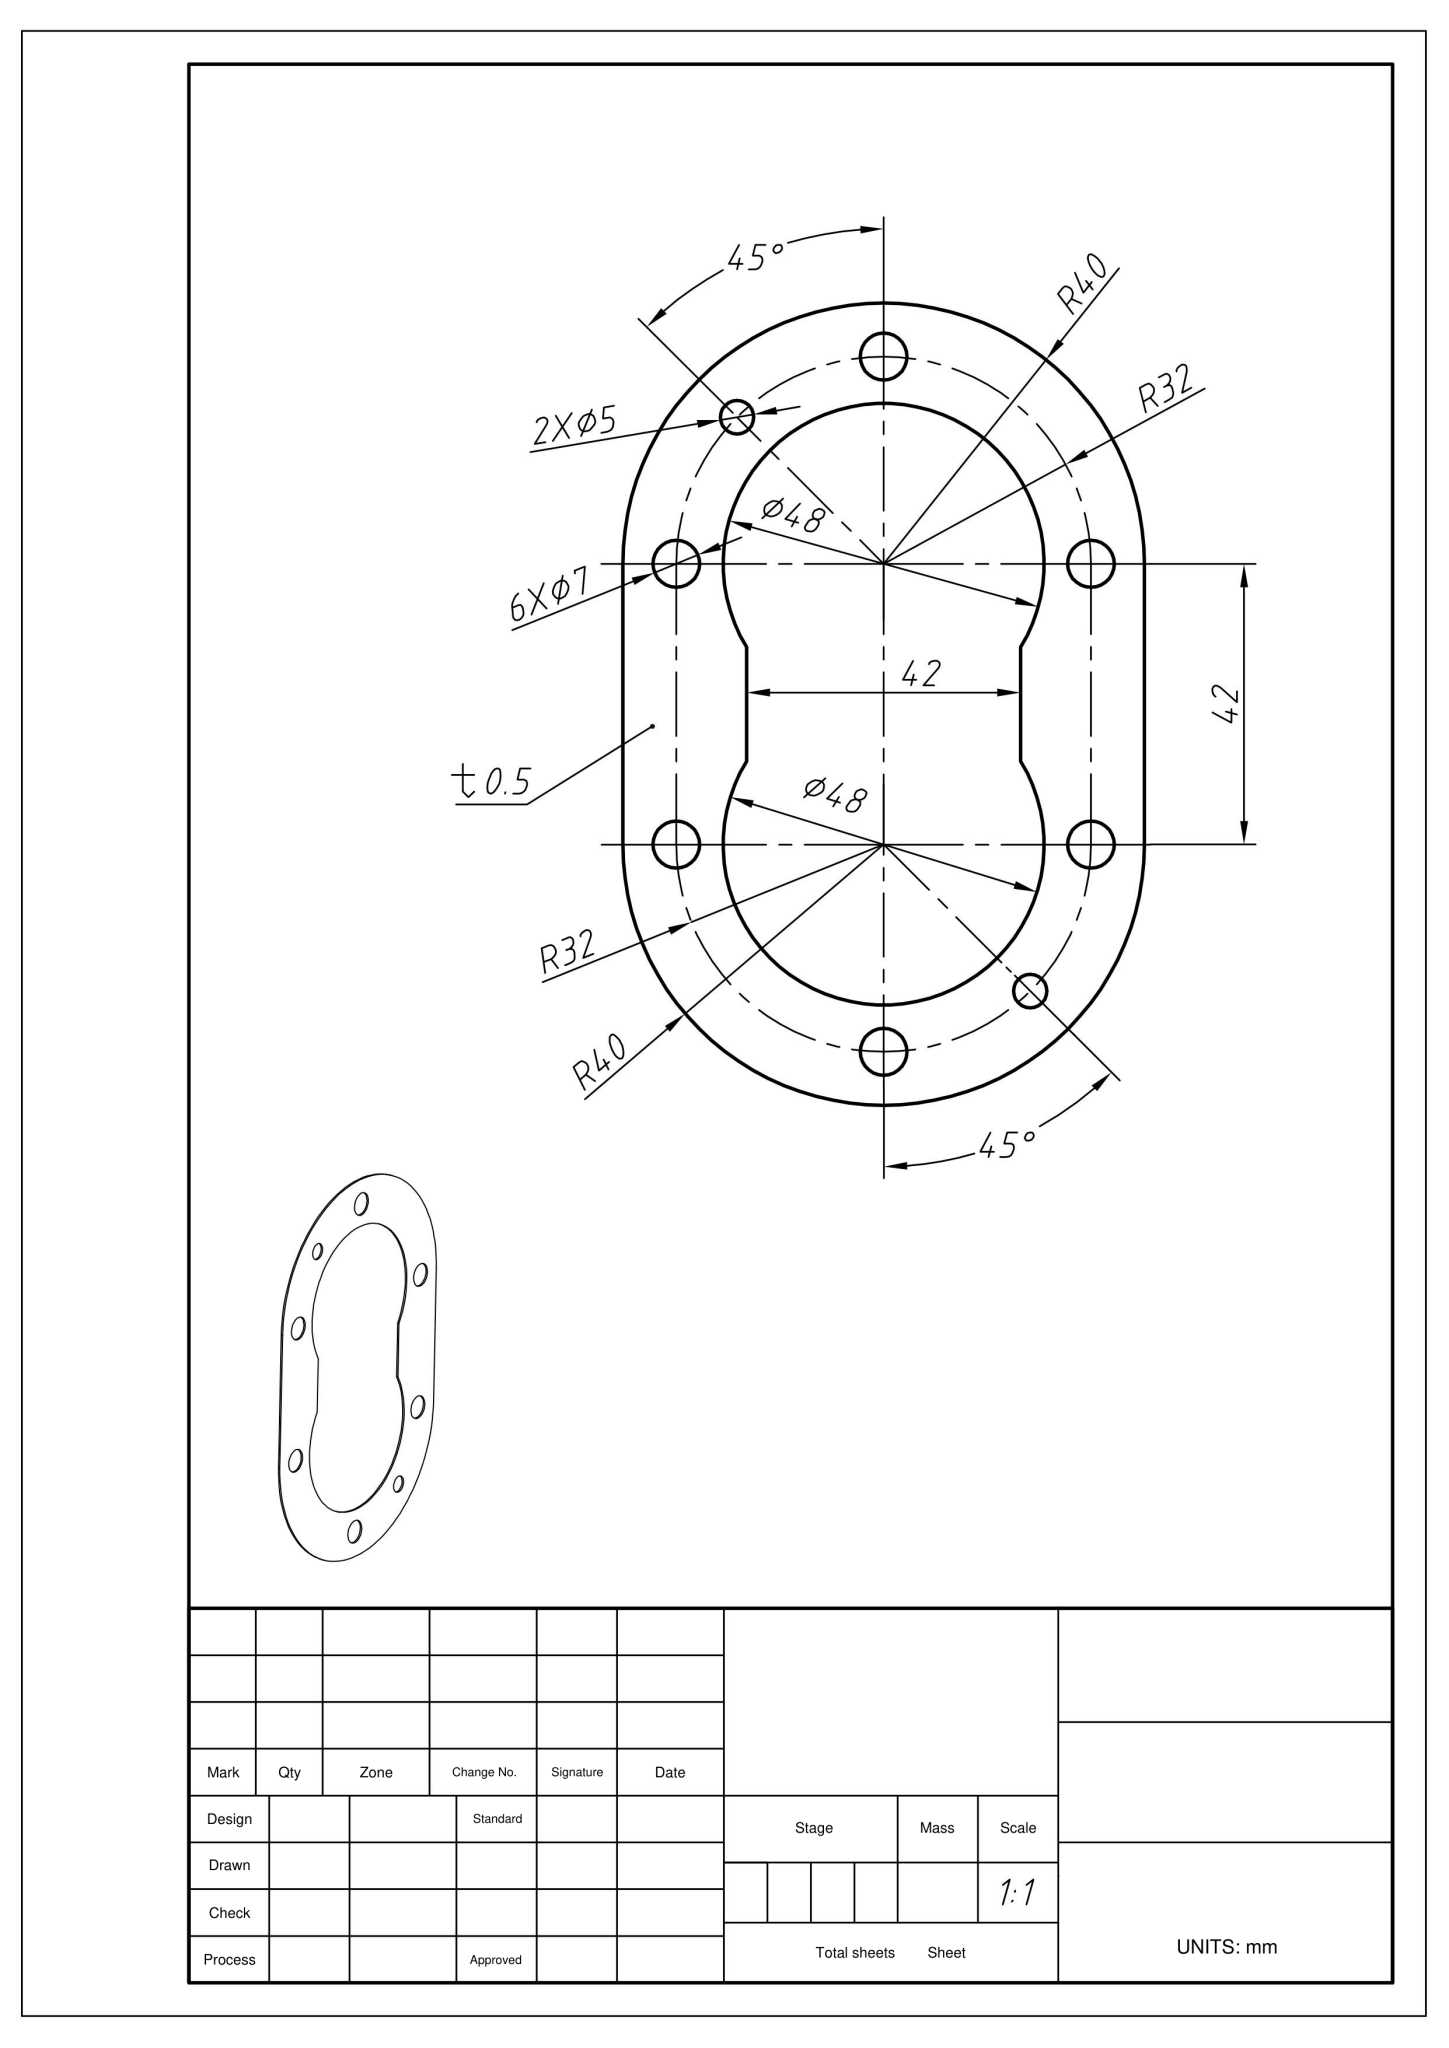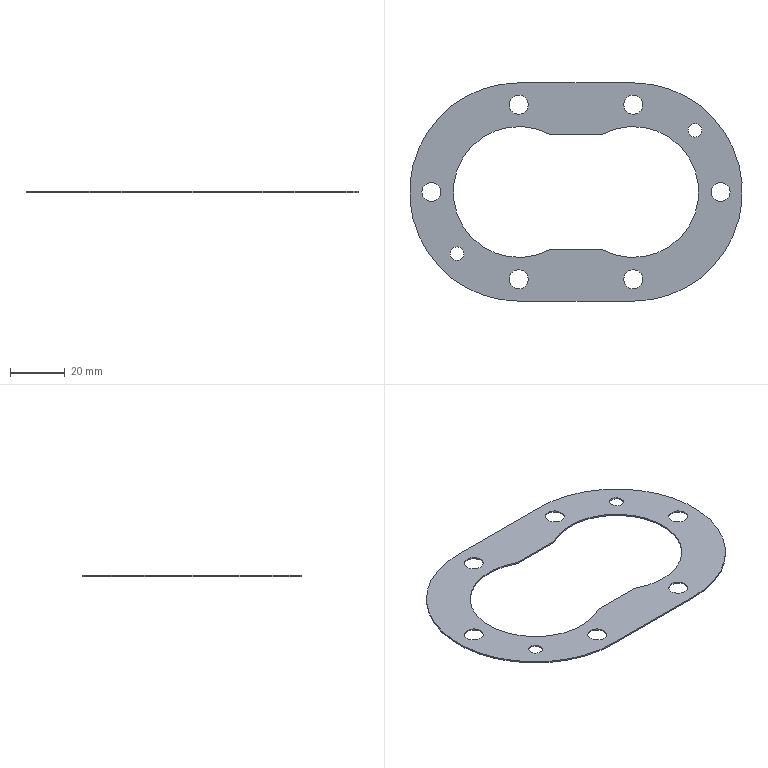Part | NX | mm | 1 solid | 18 faces | box 122 x 80 x 0.5 mm | volume 2224 mm3 | cylinder 12 | plane 6 | commonest cylinder face diameters 7 x6 48 x2 80 x2 5 x2
STEP:
#1=CARTESIAN_POINT('',(0.,0.,0.));
#2=DIRECTION('',(0.,0.,1.));
#3=DIRECTION('',(1.,0.,0.));
#4=AXIS2_PLACEMENT_3D('',#1,#2,#3);
#5=(LENGTH_UNIT()NAMED_UNIT(*)SI_UNIT(.MILLI.,.METRE.));
#6=UNCERTAINTY_MEASURE_WITH_UNIT(LENGTH_MEASURE(0.00002),#5,'','');
#7=(NAMED_UNIT(*)PLANE_ANGLE_UNIT()SI_UNIT($,.RADIAN.));
#8=PLANE_ANGLE_MEASURE_WITH_UNIT(PLANE_ANGLE_MEASURE(0.01745),#7);
#9=DIMENSIONAL_EXPONENTS(0.,0.,0.,0.,0.,0.,0.);
#10=(CONVERSION_BASED_UNIT('',#8)NAMED_UNIT(#9)PLANE_ANGLE_UNIT());
#11=(NAMED_UNIT(*)SI_UNIT($,.STERADIAN.)SOLID_ANGLE_UNIT());
#12=(GEOMETRIC_REPRESENTATION_CONTEXT(3)GLOBAL_UNCERTAINTY_ASSIGNED_CONTEXT((#6))GLOBAL_UNIT_ASSIGNED_CONTEXT((#5,#10,#11))REPRESENTATION_CONTEXT('',''));
#13=SHAPE_REPRESENTATION('',(#4),#12);
#14=CARTESIAN_POINT('',(-9.381,-21.,0.));
#15=VERTEX_POINT('',#14);
#16=CARTESIAN_POINT('',(-9.381,21.,0.));
#17=VERTEX_POINT('',#16);
#18=CARTESIAN_POINT('',(-21.,0.,0.));
#19=DIRECTION('',(0.,0.,-1.));
#20=DIRECTION('',(0.,-1.,0.));
#21=AXIS2_PLACEMENT_3D('',#18,#19,#20);
#22=CIRCLE('',#21,24.);
#23=EDGE_CURVE('',#15,#17,#22,.T.);
#24=ORIENTED_EDGE('',*,*,#23,.F.);
#25=CARTESIAN_POINT('',(-9.381,-21.,-0.5));
#26=VERTEX_POINT('',#25);
#27=CARTESIAN_POINT('',(-9.381,-21.,-0.5));
#28=DIRECTION('',(0.,0.,1.));
#29=VECTOR('',#28,1.);
#30=LINE('',#27,#29);
#31=EDGE_CURVE('',#26,#15,#30,.T.);
#32=ORIENTED_EDGE('',*,*,#31,.F.);
#33=CARTESIAN_POINT('',(-9.381,21.,-0.5));
#34=VERTEX_POINT('',#33);
#35=CARTESIAN_POINT('',(-21.,0.,-0.5));
#36=DIRECTION('',(0.,0.,-1.));
#37=DIRECTION('',(0.,-1.,0.));
#38=AXIS2_PLACEMENT_3D('',#35,#36,#37);
#39=CIRCLE('',#38,24.);
#40=EDGE_CURVE('',#26,#34,#39,.T.);
#41=ORIENTED_EDGE('',*,*,#40,.T.);
#42=CARTESIAN_POINT('',(-9.381,21.,-0.5));
#43=DIRECTION('',(0.,0.,1.));
#44=VECTOR('',#43,1.);
#45=LINE('',#42,#44);
#46=EDGE_CURVE('',#34,#17,#45,.T.);
#47=ORIENTED_EDGE('',*,*,#46,.T.);
#48=EDGE_LOOP('',(#24,#32,#41,#47));
#49=FACE_OUTER_BOUND('',#48,.T.);
#50=CARTESIAN_POINT('',(-21.,0.,-0.5));
#51=DIRECTION('',(0.,0.,1.));
#52=DIRECTION('',(1.,0.,0.));
#53=AXIS2_PLACEMENT_3D('',#50,#51,#52);
#54=CYLINDRICAL_SURFACE('',#53,24.);
#55=ADVANCED_FACE('',(#49),#54,.F.);
#56=CARTESIAN_POINT('',(9.381,21.,0.));
#57=VERTEX_POINT('',#56);
#58=CARTESIAN_POINT('',(-9.381,21.,0.));
#59=DIRECTION('',(1.,0.,0.));
#60=VECTOR('',#59,1.);
#61=LINE('',#58,#60);
#62=EDGE_CURVE('',#17,#57,#61,.T.);
#63=ORIENTED_EDGE('',*,*,#62,.F.);
#64=ORIENTED_EDGE('',*,*,#46,.F.);
#65=CARTESIAN_POINT('',(9.381,21.,-0.5));
#66=VERTEX_POINT('',#65);
#67=CARTESIAN_POINT('',(-9.381,21.,-0.5));
#68=DIRECTION('',(1.,0.,0.));
#69=VECTOR('',#68,1.);
#70=LINE('',#67,#69);
#71=EDGE_CURVE('',#34,#66,#70,.T.);
#72=ORIENTED_EDGE('',*,*,#71,.T.);
#73=CARTESIAN_POINT('',(9.381,21.,-0.5));
#74=DIRECTION('',(0.,0.,1.));
#75=VECTOR('',#74,1.);
#76=LINE('',#73,#75);
#77=EDGE_CURVE('',#66,#57,#76,.T.);
#78=ORIENTED_EDGE('',*,*,#77,.T.);
#79=EDGE_LOOP('',(#63,#64,#72,#78));
#80=FACE_OUTER_BOUND('',#79,.T.);
#81=CARTESIAN_POINT('',(-9.381,21.,-0.5));
#82=DIRECTION('',(0.,-1.,0.));
#83=DIRECTION('',(0.,0.,-1.));
#84=AXIS2_PLACEMENT_3D('',#81,#82,#83);
#85=PLANE('',#84);
#86=ADVANCED_FACE('',(#80),#85,.T.);
#87=CARTESIAN_POINT('',(9.381,-21.,0.));
#88=VERTEX_POINT('',#87);
#89=CARTESIAN_POINT('',(21.,0.,0.));
#90=DIRECTION('',(0.,0.,-1.));
#91=DIRECTION('',(0.,-1.,0.));
#92=AXIS2_PLACEMENT_3D('',#89,#90,#91);
#93=CIRCLE('',#92,24.);
#94=EDGE_CURVE('',#57,#88,#93,.T.);
#95=ORIENTED_EDGE('',*,*,#94,.F.);
#96=ORIENTED_EDGE('',*,*,#77,.F.);
#97=CARTESIAN_POINT('',(9.381,-21.,-0.5));
#98=VERTEX_POINT('',#97);
#99=CARTESIAN_POINT('',(21.,0.,-0.5));
#100=DIRECTION('',(0.,0.,-1.));
#101=DIRECTION('',(0.,-1.,0.));
#102=AXIS2_PLACEMENT_3D('',#99,#100,#101);
#103=CIRCLE('',#102,24.);
#104=EDGE_CURVE('',#66,#98,#103,.T.);
#105=ORIENTED_EDGE('',*,*,#104,.T.);
#106=CARTESIAN_POINT('',(9.381,-21.,-0.5));
#107=DIRECTION('',(0.,0.,1.));
#108=VECTOR('',#107,1.);
#109=LINE('',#106,#108);
#110=EDGE_CURVE('',#98,#88,#109,.T.);
#111=ORIENTED_EDGE('',*,*,#110,.T.);
#112=EDGE_LOOP('',(#95,#96,#105,#111));
#113=FACE_OUTER_BOUND('',#112,.T.);
#114=CARTESIAN_POINT('',(21.,0.,-0.5));
#115=DIRECTION('',(0.,0.,1.));
#116=DIRECTION('',(1.,0.,0.));
#117=AXIS2_PLACEMENT_3D('',#114,#115,#116);
#118=CYLINDRICAL_SURFACE('',#117,24.);
#119=ADVANCED_FACE('',(#113),#118,.F.);
#120=CARTESIAN_POINT('',(-21.,40.,0.));
#121=VERTEX_POINT('',#120);
#122=CARTESIAN_POINT('',(-21.,-40.,0.));
#123=VERTEX_POINT('',#122);
#124=CARTESIAN_POINT('',(-21.,0.,0.));
#125=DIRECTION('',(0.,0.,1.));
#126=DIRECTION('',(-0.,-1.,0.));
#127=AXIS2_PLACEMENT_3D('',#124,#125,#126);
#128=CIRCLE('',#127,40.);
#129=EDGE_CURVE('',#121,#123,#128,.T.);
#130=ORIENTED_EDGE('',*,*,#129,.F.);
#131=CARTESIAN_POINT('',(-21.,40.,-0.5));
#132=VERTEX_POINT('',#131);
#133=CARTESIAN_POINT('',(-21.,40.,-0.5));
#134=DIRECTION('',(0.,0.,1.));
#135=VECTOR('',#134,1.);
#136=LINE('',#133,#135);
#137=EDGE_CURVE('',#132,#121,#136,.T.);
#138=ORIENTED_EDGE('',*,*,#137,.F.);
#139=CARTESIAN_POINT('',(-21.,-40.,-0.5));
#140=VERTEX_POINT('',#139);
#141=CARTESIAN_POINT('',(-21.,0.,-0.5));
#142=DIRECTION('',(0.,0.,1.));
#143=DIRECTION('',(-0.,-1.,0.));
#144=AXIS2_PLACEMENT_3D('',#141,#142,#143);
#145=CIRCLE('',#144,40.);
#146=EDGE_CURVE('',#132,#140,#145,.T.);
#147=ORIENTED_EDGE('',*,*,#146,.T.);
#148=CARTESIAN_POINT('',(-21.,-40.,-0.5));
#149=DIRECTION('',(0.,0.,1.));
#150=VECTOR('',#149,1.);
#151=LINE('',#148,#150);
#152=EDGE_CURVE('',#140,#123,#151,.T.);
#153=ORIENTED_EDGE('',*,*,#152,.T.);
#154=EDGE_LOOP('',(#130,#138,#147,#153));
#155=FACE_OUTER_BOUND('',#154,.T.);
#156=CARTESIAN_POINT('',(-21.,0.,-0.5));
#157=DIRECTION('',(0.,0.,1.));
#158=DIRECTION('',(1.,0.,0.));
#159=AXIS2_PLACEMENT_3D('',#156,#157,#158);
#160=CYLINDRICAL_SURFACE('',#159,40.);
#161=ADVANCED_FACE('',(#155),#160,.T.);
#162=CARTESIAN_POINT('',(21.,-40.,0.));
#163=VERTEX_POINT('',#162);
#164=CARTESIAN_POINT('',(-21.,-40.,0.));
#165=DIRECTION('',(1.,-0.,0.));
#166=VECTOR('',#165,1.);
#167=LINE('',#164,#166);
#168=EDGE_CURVE('',#123,#163,#167,.T.);
#169=ORIENTED_EDGE('',*,*,#168,.F.);
#170=ORIENTED_EDGE('',*,*,#152,.F.);
#171=CARTESIAN_POINT('',(21.,-40.,-0.5));
#172=VERTEX_POINT('',#171);
#173=CARTESIAN_POINT('',(-21.,-40.,-0.5));
#174=DIRECTION('',(1.,-0.,0.));
#175=VECTOR('',#174,1.);
#176=LINE('',#173,#175);
#177=EDGE_CURVE('',#140,#172,#176,.T.);
#178=ORIENTED_EDGE('',*,*,#177,.T.);
#179=CARTESIAN_POINT('',(21.,-40.,-0.5));
#180=DIRECTION('',(0.,0.,1.));
#181=VECTOR('',#180,1.);
#182=LINE('',#179,#181);
#183=EDGE_CURVE('',#172,#163,#182,.T.);
#184=ORIENTED_EDGE('',*,*,#183,.T.);
#185=EDGE_LOOP('',(#169,#170,#178,#184));
#186=FACE_OUTER_BOUND('',#185,.T.);
#187=CARTESIAN_POINT('',(-21.,-40.,-0.5));
#188=DIRECTION('',(-0.,-1.,0.));
#189=DIRECTION('',(1.,-0.,0.));
#190=AXIS2_PLACEMENT_3D('',#187,#188,#189);
#191=PLANE('',#190);
#192=ADVANCED_FACE('',(#186),#191,.T.);
#193=CARTESIAN_POINT('',(21.,40.,0.));
#194=VERTEX_POINT('',#193);
#195=CARTESIAN_POINT('',(21.,0.,0.));
#196=DIRECTION('',(0.,0.,1.));
#197=DIRECTION('',(-0.,-1.,0.));
#198=AXIS2_PLACEMENT_3D('',#195,#196,#197);
#199=CIRCLE('',#198,40.);
#200=EDGE_CURVE('',#163,#194,#199,.T.);
#201=ORIENTED_EDGE('',*,*,#200,.F.);
#202=ORIENTED_EDGE('',*,*,#183,.F.);
#203=CARTESIAN_POINT('',(21.,40.,-0.5));
#204=VERTEX_POINT('',#203);
#205=CARTESIAN_POINT('',(21.,0.,-0.5));
#206=DIRECTION('',(0.,0.,1.));
#207=DIRECTION('',(-0.,-1.,0.));
#208=AXIS2_PLACEMENT_3D('',#205,#206,#207);
#209=CIRCLE('',#208,40.);
#210=EDGE_CURVE('',#172,#204,#209,.T.);
#211=ORIENTED_EDGE('',*,*,#210,.T.);
#212=CARTESIAN_POINT('',(21.,40.,-0.5));
#213=DIRECTION('',(0.,0.,1.));
#214=VECTOR('',#213,1.);
#215=LINE('',#212,#214);
#216=EDGE_CURVE('',#204,#194,#215,.T.);
#217=ORIENTED_EDGE('',*,*,#216,.T.);
#218=EDGE_LOOP('',(#201,#202,#211,#217));
#219=FACE_OUTER_BOUND('',#218,.T.);
#220=CARTESIAN_POINT('',(21.,0.,-0.5));
#221=DIRECTION('',(0.,0.,1.));
#222=DIRECTION('',(1.,0.,0.));
#223=AXIS2_PLACEMENT_3D('',#220,#221,#222);
#224=CYLINDRICAL_SURFACE('',#223,40.);
#225=ADVANCED_FACE('',(#219),#224,.T.);
#226=CARTESIAN_POINT('',(56.5,-0.,-0.5));
#227=VERTEX_POINT('',#226);
#228=CARTESIAN_POINT('',(53.,-0.,-0.5));
#229=DIRECTION('',(0.,0.,1.));
#230=DIRECTION('',(1.,0.,0.));
#231=AXIS2_PLACEMENT_3D('',#228,#229,#230);
#232=CIRCLE('',#231,3.5);
#233=EDGE_CURVE('',#227,#227,#232,.T.);
#234=ORIENTED_EDGE('',*,*,#233,.F.);
#235=EDGE_LOOP('',(#234));
#236=FACE_BOUND('',#235,.T.);
#237=CARTESIAN_POINT('',(56.5,-0.,0.));
#238=VERTEX_POINT('',#237);
#239=CARTESIAN_POINT('',(53.,-0.,0.));
#240=DIRECTION('',(0.,0.,1.));
#241=DIRECTION('',(1.,0.,0.));
#242=AXIS2_PLACEMENT_3D('',#239,#240,#241);
#243=CIRCLE('',#242,3.5);
#244=EDGE_CURVE('',#238,#238,#243,.T.);
#245=ORIENTED_EDGE('',*,*,#244,.T.);
#246=EDGE_LOOP('',(#245));
#247=FACE_BOUND('',#246,.T.);
#248=CARTESIAN_POINT('',(53.,-0.,-0.5));
#249=DIRECTION('',(0.,0.,1.));
#250=DIRECTION('',(1.,0.,0.));
#251=AXIS2_PLACEMENT_3D('',#248,#249,#250);
#252=CYLINDRICAL_SURFACE('',#251,3.5);
#253=ADVANCED_FACE('',(#236,#247),#252,.F.);
#254=CARTESIAN_POINT('',(43.627,20.127,-0.5));
#255=VERTEX_POINT('',#254);
#256=CARTESIAN_POINT('',(43.627,22.627,-0.5));
#257=DIRECTION('',(0.,0.,1.));
#258=DIRECTION('',(0.,-1.,0.));
#259=AXIS2_PLACEMENT_3D('',#256,#257,#258);
#260=CIRCLE('',#259,2.5);
#261=EDGE_CURVE('',#255,#255,#260,.T.);
#262=ORIENTED_EDGE('',*,*,#261,.F.);
#263=EDGE_LOOP('',(#262));
#264=FACE_BOUND('',#263,.T.);
#265=CARTESIAN_POINT('',(43.627,20.127,0.));
#266=VERTEX_POINT('',#265);
#267=CARTESIAN_POINT('',(43.627,22.627,0.));
#268=DIRECTION('',(0.,0.,1.));
#269=DIRECTION('',(0.,-1.,0.));
#270=AXIS2_PLACEMENT_3D('',#267,#268,#269);
#271=CIRCLE('',#270,2.5);
#272=EDGE_CURVE('',#266,#266,#271,.T.);
#273=ORIENTED_EDGE('',*,*,#272,.T.);
#274=EDGE_LOOP('',(#273));
#275=FACE_BOUND('',#274,.T.);
#276=CARTESIAN_POINT('',(43.627,22.627,-0.5));
#277=DIRECTION('',(0.,0.,1.));
#278=DIRECTION('',(1.,0.,0.));
#279=AXIS2_PLACEMENT_3D('',#276,#277,#278);
#280=CYLINDRICAL_SURFACE('',#279,2.5);
#281=ADVANCED_FACE('',(#264,#275),#280,.F.);
#282=CARTESIAN_POINT('',(21.,35.5,-0.5));
#283=VERTEX_POINT('',#282);
#284=CARTESIAN_POINT('',(21.,32.,-0.5));
#285=DIRECTION('',(0.,0.,1.));
#286=DIRECTION('',(0.,1.,0.));
#287=AXIS2_PLACEMENT_3D('',#284,#285,#286);
#288=CIRCLE('',#287,3.5);
#289=EDGE_CURVE('',#283,#283,#288,.T.);
#290=ORIENTED_EDGE('',*,*,#289,.F.);
#291=EDGE_LOOP('',(#290));
#292=FACE_BOUND('',#291,.T.);
#293=CARTESIAN_POINT('',(21.,35.5,0.));
#294=VERTEX_POINT('',#293);
#295=CARTESIAN_POINT('',(21.,32.,0.));
#296=DIRECTION('',(0.,0.,1.));
#297=DIRECTION('',(0.,1.,0.));
#298=AXIS2_PLACEMENT_3D('',#295,#296,#297);
#299=CIRCLE('',#298,3.5);
#300=EDGE_CURVE('',#294,#294,#299,.T.);
#301=ORIENTED_EDGE('',*,*,#300,.T.);
#302=EDGE_LOOP('',(#301));
#303=FACE_BOUND('',#302,.T.);
#304=CARTESIAN_POINT('',(21.,32.,-0.5));
#305=DIRECTION('',(0.,0.,1.));
#306=DIRECTION('',(1.,0.,0.));
#307=AXIS2_PLACEMENT_3D('',#304,#305,#306);
#308=CYLINDRICAL_SURFACE('',#307,3.5);
#309=ADVANCED_FACE('',(#292,#303),#308,.F.);
#310=CARTESIAN_POINT('',(21.,-35.5,-0.5));
#311=VERTEX_POINT('',#310);
#312=CARTESIAN_POINT('',(21.,-32.,-0.5));
#313=DIRECTION('',(0.,0.,1.));
#314=DIRECTION('',(0.,-1.,0.));
#315=AXIS2_PLACEMENT_3D('',#312,#313,#314);
#316=CIRCLE('',#315,3.5);
#317=EDGE_CURVE('',#311,#311,#316,.T.);
#318=ORIENTED_EDGE('',*,*,#317,.F.);
#319=EDGE_LOOP('',(#318));
#320=FACE_BOUND('',#319,.T.);
#321=CARTESIAN_POINT('',(21.,-35.5,0.));
#322=VERTEX_POINT('',#321);
#323=CARTESIAN_POINT('',(21.,-32.,0.));
#324=DIRECTION('',(0.,0.,1.));
#325=DIRECTION('',(0.,-1.,0.));
#326=AXIS2_PLACEMENT_3D('',#323,#324,#325);
#327=CIRCLE('',#326,3.5);
#328=EDGE_CURVE('',#322,#322,#327,.T.);
#329=ORIENTED_EDGE('',*,*,#328,.T.);
#330=EDGE_LOOP('',(#329));
#331=FACE_BOUND('',#330,.T.);
#332=CARTESIAN_POINT('',(21.,-32.,-0.5));
#333=DIRECTION('',(0.,0.,1.));
#334=DIRECTION('',(1.,0.,0.));
#335=AXIS2_PLACEMENT_3D('',#332,#333,#334);
#336=CYLINDRICAL_SURFACE('',#335,3.5);
#337=ADVANCED_FACE('',(#320,#331),#336,.F.);
#338=CARTESIAN_POINT('',(-21.,-35.5,-0.5));
#339=VERTEX_POINT('',#338);
#340=CARTESIAN_POINT('',(-21.,-32.,-0.5));
#341=DIRECTION('',(0.,0.,-1.));
#342=DIRECTION('',(0.,-1.,0.));
#343=AXIS2_PLACEMENT_3D('',#340,#341,#342);
#344=CIRCLE('',#343,3.5);
#345=EDGE_CURVE('',#339,#339,#344,.T.);
#346=ORIENTED_EDGE('',*,*,#345,.T.);
#347=EDGE_LOOP('',(#346));
#348=FACE_BOUND('',#347,.T.);
#349=CARTESIAN_POINT('',(-21.,-35.5,0.));
#350=VERTEX_POINT('',#349);
#351=CARTESIAN_POINT('',(-21.,-32.,0.));
#352=DIRECTION('',(0.,0.,-1.));
#353=DIRECTION('',(0.,-1.,0.));
#354=AXIS2_PLACEMENT_3D('',#351,#352,#353);
#355=CIRCLE('',#354,3.5);
#356=EDGE_CURVE('',#350,#350,#355,.T.);
#357=ORIENTED_EDGE('',*,*,#356,.F.);
#358=EDGE_LOOP('',(#357));
#359=FACE_BOUND('',#358,.T.);
#360=CARTESIAN_POINT('',(-21.,-32.,-0.5));
#361=DIRECTION('',(0.,0.,1.));
#362=DIRECTION('',(1.,0.,0.));
#363=AXIS2_PLACEMENT_3D('',#360,#361,#362);
#364=CYLINDRICAL_SURFACE('',#363,3.5);
#365=ADVANCED_FACE('',(#348,#359),#364,.F.);
#366=CARTESIAN_POINT('',(-43.627,-25.127,-0.5));
#367=VERTEX_POINT('',#366);
#368=CARTESIAN_POINT('',(-43.627,-22.627,-0.5));
#369=DIRECTION('',(0.,0.,1.));
#370=DIRECTION('',(0.,-1.,0.));
#371=AXIS2_PLACEMENT_3D('',#368,#369,#370);
#372=CIRCLE('',#371,2.5);
#373=EDGE_CURVE('',#367,#367,#372,.T.);
#374=ORIENTED_EDGE('',*,*,#373,.F.);
#375=EDGE_LOOP('',(#374));
#376=FACE_BOUND('',#375,.T.);
#377=CARTESIAN_POINT('',(-43.627,-25.127,0.));
#378=VERTEX_POINT('',#377);
#379=CARTESIAN_POINT('',(-43.627,-22.627,0.));
#380=DIRECTION('',(0.,0.,1.));
#381=DIRECTION('',(0.,-1.,0.));
#382=AXIS2_PLACEMENT_3D('',#379,#380,#381);
#383=CIRCLE('',#382,2.5);
#384=EDGE_CURVE('',#378,#378,#383,.T.);
#385=ORIENTED_EDGE('',*,*,#384,.T.);
#386=EDGE_LOOP('',(#385));
#387=FACE_BOUND('',#386,.T.);
#388=CARTESIAN_POINT('',(-43.627,-22.627,-0.5));
#389=DIRECTION('',(0.,0.,1.));
#390=DIRECTION('',(1.,0.,0.));
#391=AXIS2_PLACEMENT_3D('',#388,#389,#390);
#392=CYLINDRICAL_SURFACE('',#391,2.5);
#393=ADVANCED_FACE('',(#376,#387),#392,.F.);
#394=CARTESIAN_POINT('',(-56.5,-0.,-0.5));
#395=VERTEX_POINT('',#394);
#396=CARTESIAN_POINT('',(-53.,-0.,-0.5));
#397=DIRECTION('',(0.,0.,-1.));
#398=DIRECTION('',(-1.,0.,0.));
#399=AXIS2_PLACEMENT_3D('',#396,#397,#398);
#400=CIRCLE('',#399,3.5);
#401=EDGE_CURVE('',#395,#395,#400,.T.);
#402=ORIENTED_EDGE('',*,*,#401,.T.);
#403=EDGE_LOOP('',(#402));
#404=FACE_BOUND('',#403,.T.);
#405=CARTESIAN_POINT('',(-56.5,-0.,0.));
#406=VERTEX_POINT('',#405);
#407=CARTESIAN_POINT('',(-53.,-0.,0.));
#408=DIRECTION('',(0.,0.,-1.));
#409=DIRECTION('',(-1.,0.,0.));
#410=AXIS2_PLACEMENT_3D('',#407,#408,#409);
#411=CIRCLE('',#410,3.5);
#412=EDGE_CURVE('',#406,#406,#411,.T.);
#413=ORIENTED_EDGE('',*,*,#412,.F.);
#414=EDGE_LOOP('',(#413));
#415=FACE_BOUND('',#414,.T.);
#416=CARTESIAN_POINT('',(-53.,-0.,-0.5));
#417=DIRECTION('',(0.,0.,1.));
#418=DIRECTION('',(1.,0.,0.));
#419=AXIS2_PLACEMENT_3D('',#416,#417,#418);
#420=CYLINDRICAL_SURFACE('',#419,3.5);
#421=ADVANCED_FACE('',(#404,#415),#420,.F.);
#422=CARTESIAN_POINT('',(-21.,35.5,-0.5));
#423=VERTEX_POINT('',#422);
#424=CARTESIAN_POINT('',(-21.,32.,-0.5));
#425=DIRECTION('',(0.,0.,-1.));
#426=DIRECTION('',(0.,1.,0.));
#427=AXIS2_PLACEMENT_3D('',#424,#425,#426);
#428=CIRCLE('',#427,3.5);
#429=EDGE_CURVE('',#423,#423,#428,.T.);
#430=ORIENTED_EDGE('',*,*,#429,.T.);
#431=EDGE_LOOP('',(#430));
#432=FACE_BOUND('',#431,.T.);
#433=CARTESIAN_POINT('',(-21.,35.5,0.));
#434=VERTEX_POINT('',#433);
#435=CARTESIAN_POINT('',(-21.,32.,0.));
#436=DIRECTION('',(0.,0.,-1.));
#437=DIRECTION('',(0.,1.,0.));
#438=AXIS2_PLACEMENT_3D('',#435,#436,#437);
#439=CIRCLE('',#438,3.5);
#440=EDGE_CURVE('',#434,#434,#439,.T.);
#441=ORIENTED_EDGE('',*,*,#440,.F.);
#442=EDGE_LOOP('',(#441));
#443=FACE_BOUND('',#442,.T.);
#444=CARTESIAN_POINT('',(-21.,32.,-0.5));
#445=DIRECTION('',(0.,0.,1.));
#446=DIRECTION('',(1.,0.,0.));
#447=AXIS2_PLACEMENT_3D('',#444,#445,#446);
#448=CYLINDRICAL_SURFACE('',#447,3.5);
#449=ADVANCED_FACE('',(#432,#443),#448,.F.);
#450=CARTESIAN_POINT('',(21.,40.,0.));
#451=DIRECTION('',(-1.,0.,0.));
#452=VECTOR('',#451,1.);
#453=LINE('',#450,#452);
#454=EDGE_CURVE('',#194,#121,#453,.T.);
#455=ORIENTED_EDGE('',*,*,#454,.F.);
#456=ORIENTED_EDGE('',*,*,#216,.F.);
#457=CARTESIAN_POINT('',(21.,40.,-0.5));
#458=DIRECTION('',(-1.,0.,0.));
#459=VECTOR('',#458,1.);
#460=LINE('',#457,#459);
#461=EDGE_CURVE('',#204,#132,#460,.T.);
#462=ORIENTED_EDGE('',*,*,#461,.T.);
#463=ORIENTED_EDGE('',*,*,#137,.T.);
#464=EDGE_LOOP('',(#455,#456,#462,#463));
#465=FACE_OUTER_BOUND('',#464,.T.);
#466=CARTESIAN_POINT('',(21.,40.,-0.5));
#467=DIRECTION('',(0.,1.,0.));
#468=DIRECTION('',(-1.,0.,0.));
#469=AXIS2_PLACEMENT_3D('',#466,#467,#468);
#470=PLANE('',#469);
#471=ADVANCED_FACE('',(#465),#470,.T.);
#472=CARTESIAN_POINT('',(9.381,-21.,0.));
#473=DIRECTION('',(-1.,-0.,0.));
#474=VECTOR('',#473,1.);
#475=LINE('',#472,#474);
#476=EDGE_CURVE('',#88,#15,#475,.T.);
#477=ORIENTED_EDGE('',*,*,#476,.F.);
#478=ORIENTED_EDGE('',*,*,#110,.F.);
#479=CARTESIAN_POINT('',(9.381,-21.,-0.5));
#480=DIRECTION('',(-1.,-0.,0.));
#481=VECTOR('',#480,1.);
#482=LINE('',#479,#481);
#483=EDGE_CURVE('',#98,#26,#482,.T.);
#484=ORIENTED_EDGE('',*,*,#483,.T.);
#485=ORIENTED_EDGE('',*,*,#31,.T.);
#486=EDGE_LOOP('',(#477,#478,#484,#485));
#487=FACE_OUTER_BOUND('',#486,.T.);
#488=CARTESIAN_POINT('',(9.381,-21.,-0.5));
#489=DIRECTION('',(-0.,1.,0.));
#490=DIRECTION('',(-1.,-0.,0.));
#491=AXIS2_PLACEMENT_3D('',#488,#489,#490);
#492=PLANE('',#491);
#493=ADVANCED_FACE('',(#487),#492,.T.);
#494=ORIENTED_EDGE('',*,*,#146,.F.);
#495=ORIENTED_EDGE('',*,*,#461,.F.);
#496=ORIENTED_EDGE('',*,*,#210,.F.);
#497=ORIENTED_EDGE('',*,*,#177,.F.);
#498=EDGE_LOOP('',(#494,#495,#496,#497));
#499=FACE_BOUND('',#498,.T.);
#500=ORIENTED_EDGE('',*,*,#429,.F.);
#501=EDGE_LOOP('',(#500));
#502=FACE_BOUND('',#501,.T.);
#503=ORIENTED_EDGE('',*,*,#401,.F.);
#504=EDGE_LOOP('',(#503));
#505=FACE_BOUND('',#504,.T.);
#506=ORIENTED_EDGE('',*,*,#373,.T.);
#507=EDGE_LOOP('',(#506));
#508=FACE_BOUND('',#507,.T.);
#509=ORIENTED_EDGE('',*,*,#345,.F.);
#510=EDGE_LOOP('',(#509));
#511=FACE_BOUND('',#510,.T.);
#512=ORIENTED_EDGE('',*,*,#317,.T.);
#513=EDGE_LOOP('',(#512));
#514=FACE_BOUND('',#513,.T.);
#515=ORIENTED_EDGE('',*,*,#289,.T.);
#516=EDGE_LOOP('',(#515));
#517=FACE_BOUND('',#516,.T.);
#518=ORIENTED_EDGE('',*,*,#261,.T.);
#519=EDGE_LOOP('',(#518));
#520=FACE_BOUND('',#519,.T.);
#521=ORIENTED_EDGE('',*,*,#233,.T.);
#522=EDGE_LOOP('',(#521));
#523=FACE_BOUND('',#522,.T.);
#524=ORIENTED_EDGE('',*,*,#40,.F.);
#525=ORIENTED_EDGE('',*,*,#483,.F.);
#526=ORIENTED_EDGE('',*,*,#104,.F.);
#527=ORIENTED_EDGE('',*,*,#71,.F.);
#528=EDGE_LOOP('',(#524,#525,#526,#527));
#529=FACE_BOUND('',#528,.T.);
#530=CARTESIAN_POINT('',(-21.,0.,-0.5));
#531=DIRECTION('',(0.,0.,1.));
#532=DIRECTION('',(1.,0.,0.));
#533=AXIS2_PLACEMENT_3D('',#530,#531,#532);
#534=PLANE('',#533);
#535=ADVANCED_FACE('',(#499,#502,#505,#508,#511,#514,#517,#520,#523,#529),#534,.F.);
#536=ORIENTED_EDGE('',*,*,#129,.T.);
#537=ORIENTED_EDGE('',*,*,#168,.T.);
#538=ORIENTED_EDGE('',*,*,#200,.T.);
#539=ORIENTED_EDGE('',*,*,#454,.T.);
#540=EDGE_LOOP('',(#536,#537,#538,#539));
#541=FACE_BOUND('',#540,.T.);
#542=ORIENTED_EDGE('',*,*,#440,.T.);
#543=EDGE_LOOP('',(#542));
#544=FACE_BOUND('',#543,.T.);
#545=ORIENTED_EDGE('',*,*,#412,.T.);
#546=EDGE_LOOP('',(#545));
#547=FACE_BOUND('',#546,.T.);
#548=ORIENTED_EDGE('',*,*,#384,.F.);
#549=EDGE_LOOP('',(#548));
#550=FACE_BOUND('',#549,.T.);
#551=ORIENTED_EDGE('',*,*,#356,.T.);
#552=EDGE_LOOP('',(#551));
#553=FACE_BOUND('',#552,.T.);
#554=ORIENTED_EDGE('',*,*,#328,.F.);
#555=EDGE_LOOP('',(#554));
#556=FACE_BOUND('',#555,.T.);
#557=ORIENTED_EDGE('',*,*,#300,.F.);
#558=EDGE_LOOP('',(#557));
#559=FACE_BOUND('',#558,.T.);
#560=ORIENTED_EDGE('',*,*,#272,.F.);
#561=EDGE_LOOP('',(#560));
#562=FACE_BOUND('',#561,.T.);
#563=ORIENTED_EDGE('',*,*,#244,.F.);
#564=EDGE_LOOP('',(#563));
#565=FACE_BOUND('',#564,.T.);
#566=ORIENTED_EDGE('',*,*,#23,.T.);
#567=ORIENTED_EDGE('',*,*,#62,.T.);
#568=ORIENTED_EDGE('',*,*,#94,.T.);
#569=ORIENTED_EDGE('',*,*,#476,.T.);
#570=EDGE_LOOP('',(#566,#567,#568,#569));
#571=FACE_BOUND('',#570,.T.);
#572=CARTESIAN_POINT('',(-21.,0.,0.));
#573=DIRECTION('',(0.,0.,1.));
#574=DIRECTION('',(1.,0.,0.));
#575=AXIS2_PLACEMENT_3D('',#572,#573,#574);
#576=PLANE('',#575);
#577=ADVANCED_FACE('',(#541,#544,#547,#550,#553,#556,#559,#562,#565,#571),#576,.T.);
#578=CLOSED_SHELL('',(#55,#86,#119,#161,#192,#225,#253,#281,#309,#337,#365,#393,#421,#449,#471,#493,#535,#577));
#579=MANIFOLD_SOLID_BREP('',#578);
#580=ADVANCED_BREP_SHAPE_REPRESENTATION('',(#579),#12);
#581=SHAPE_REPRESENTATION_RELATIONSHIP('','',#13,#580);
#582=PRESENTATION_LAYER_ASSIGNMENT('','',(#579));
#583=COLOUR_RGB('',1.,0.6,0.);
#584=FILL_AREA_STYLE_COLOUR('',#583);
#585=FILL_AREA_STYLE('',(#584));
#586=SURFACE_STYLE_FILL_AREA(#585);
#587=SURFACE_SIDE_STYLE('',(#586));
#588=SURFACE_STYLE_USAGE(.BOTH.,#587);
#589=PRESENTATION_STYLE_ASSIGNMENT((#588));
#590=STYLED_ITEM('',(#589),#579);
#591=MECHANICAL_DESIGN_GEOMETRIC_PRESENTATION_REPRESENTATION('',(#590),#12);